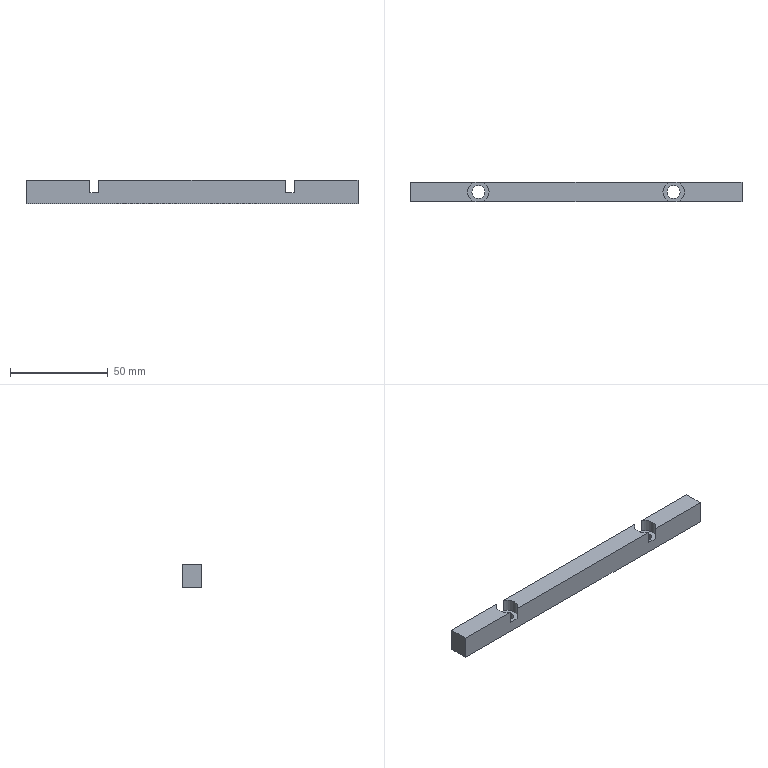Component | NX | FIXED_PLATE_10 | 1 solid | 16 faces | volume 18840 mm3 | plane 10 | cylinder 6 | commonest cylinder face diameters 11 x4 6.6 x2